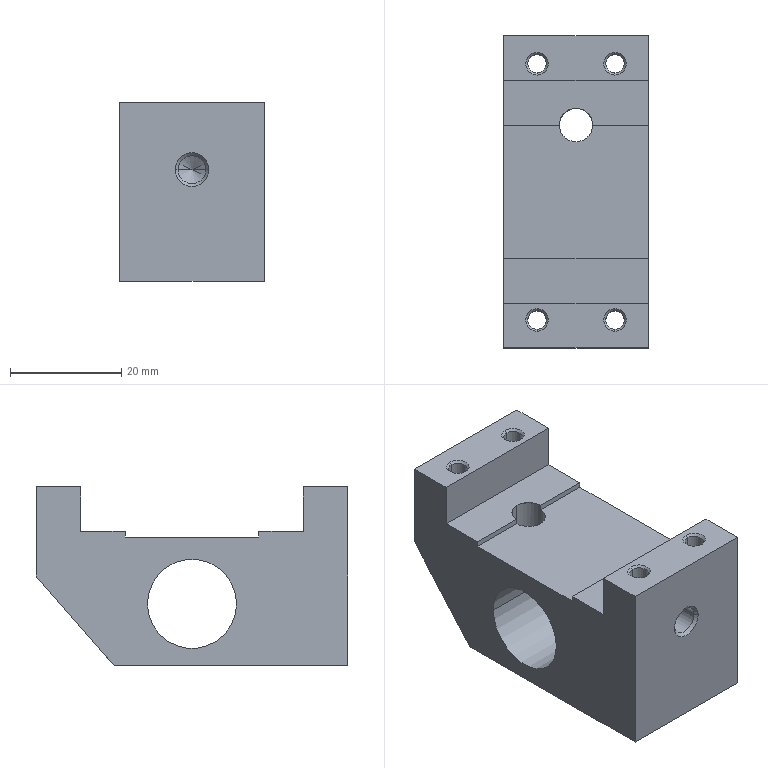Component | SolidWorks | 34Slider-1 | 1 solid | 45 faces | volume 27627 mm3 | plane 16 | cone 15 | cylinder 14 | commonest cylinder face diameters 3.3 x8 16 x2 6 x2 5 x2